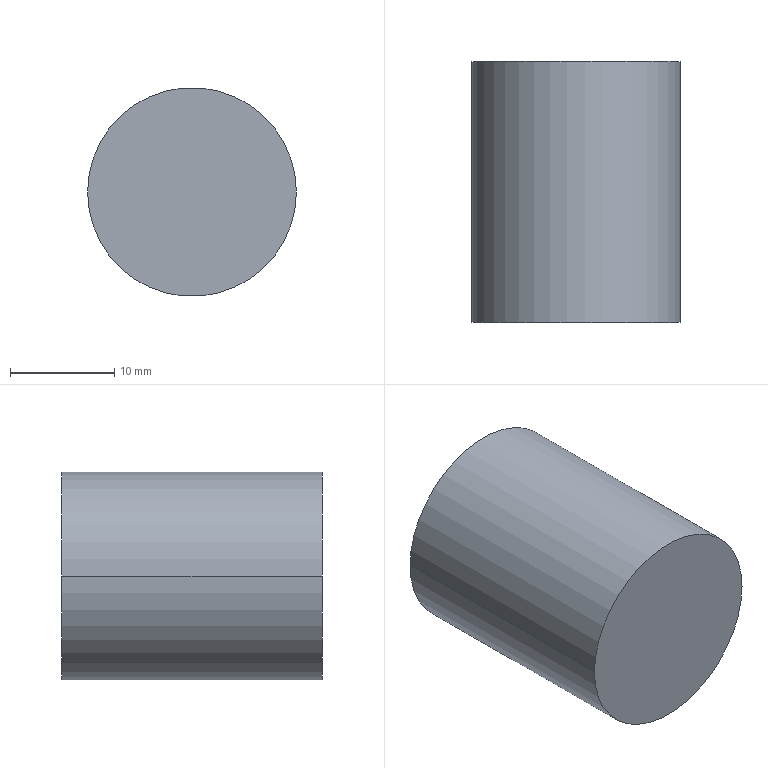Component | SolidWorks | LegSupport-1 | 1 solid | 4 faces | box 20 x 25 x 20 mm | volume 7854 mm3 | cylinder 2 | plane 2 | commonest cylinder face diameters 20 x2
build123d program:
from build123d import *

# Parameters (mm, degrees)
SKETCH1_R           = 10
BOSS_EXTRUDE1_DEPTH = 25


with BuildPart() as part:
    # Sketch1 → Boss-Extrude1 (new body)
    with BuildSketch(Plane.XY):
        with Locations((-290.265, 54.821)):
            Circle(SKETCH1_R)
    extrude(amount=BOSS_EXTRUDE1_DEPTH)


solid = part.part

# Placed as in the assembly
solid = solid.moved(Location((-81.735, 185, -108.821), (90, 0, 0)))
STEP:
#1=COLOUR_RGB('',0.7922,0.8196,0.9333);
#2=FILL_AREA_STYLE_COLOUR('',#1);
#3=FILL_AREA_STYLE('',(#2));
#4=SURFACE_STYLE_FILL_AREA(#3);
#5=SURFACE_SIDE_STYLE('',(#4));
#6=SURFACE_STYLE_USAGE(.BOTH.,#5);
#7=PRESENTATION_STYLE_ASSIGNMENT((#6));
#8=CARTESIAN_POINT('',(-14.252,7.283,-2.126));
#9=VERTEX_POINT('',#8);
#10=CARTESIAN_POINT('',(-15.039,7.283,-2.126));
#11=VERTEX_POINT('',#10);
#12=CARTESIAN_POINT('',(-14.646,7.283,-2.126));
#13=DIRECTION('',(0.,1.,0.));
#14=DIRECTION('',(1.,0.,0.));
#15=AXIS2_PLACEMENT_3D('',#12,#13,#14);
#16=CIRCLE('',#15,0.3937);
#17=EDGE_CURVE('',#9,#11,#16,.T.);
#18=ORIENTED_EDGE('',*,*,#17,.F.);
#19=CARTESIAN_POINT('',(-14.252,6.299,-2.126));
#20=VERTEX_POINT('',#19);
#21=CARTESIAN_POINT('',(-14.252,7.283,-2.126));
#22=DIRECTION('',(0.,-1.,0.));
#23=VECTOR('',#22,39.37);
#24=LINE('',#21,#23);
#25=EDGE_CURVE('',#9,#20,#24,.T.);
#26=ORIENTED_EDGE('',*,*,#25,.T.);
#27=CARTESIAN_POINT('',(-15.039,6.299,-2.126));
#28=VERTEX_POINT('',#27);
#29=CARTESIAN_POINT('',(-14.646,6.299,-2.126));
#30=DIRECTION('',(0.,1.,0.));
#31=DIRECTION('',(1.,0.,0.));
#32=AXIS2_PLACEMENT_3D('',#29,#30,#31);
#33=CIRCLE('',#32,0.3937);
#34=EDGE_CURVE('',#20,#28,#33,.T.);
#35=ORIENTED_EDGE('',*,*,#34,.T.);
#36=CARTESIAN_POINT('',(-15.039,7.283,-2.126));
#37=DIRECTION('',(0.,-1.,0.));
#38=VECTOR('',#37,39.37);
#39=LINE('',#36,#38);
#40=EDGE_CURVE('',#11,#28,#39,.T.);
#41=ORIENTED_EDGE('',*,*,#40,.F.);
#42=EDGE_LOOP('',(#18,#26,#35,#41));
#43=FACE_OUTER_BOUND('',#42,.T.);
#44=CARTESIAN_POINT('',(-14.646,7.283,-2.126));
#45=DIRECTION('',(0.,-1.,0.));
#46=DIRECTION('',(-1.,0.,0.));
#47=AXIS2_PLACEMENT_3D('',#44,#45,#46);
#48=CYLINDRICAL_SURFACE('',#47,0.3937);
#49=ADVANCED_FACE('',(#43),#48,.T.);
#50=ORIENTED_EDGE('',*,*,#25,.F.);
#51=CARTESIAN_POINT('',(-14.646,7.283,-2.126));
#52=DIRECTION('',(0.,1.,0.));
#53=DIRECTION('',(1.,0.,0.));
#54=AXIS2_PLACEMENT_3D('',#51,#52,#53);
#55=CIRCLE('',#54,0.3937);
#56=EDGE_CURVE('',#11,#9,#55,.T.);
#57=ORIENTED_EDGE('',*,*,#56,.F.);
#58=ORIENTED_EDGE('',*,*,#40,.T.);
#59=CARTESIAN_POINT('',(-14.646,6.299,-2.126));
#60=DIRECTION('',(0.,1.,0.));
#61=DIRECTION('',(1.,0.,0.));
#62=AXIS2_PLACEMENT_3D('',#59,#60,#61);
#63=CIRCLE('',#62,0.3937);
#64=EDGE_CURVE('',#28,#20,#63,.T.);
#65=ORIENTED_EDGE('',*,*,#64,.T.);
#66=EDGE_LOOP('',(#50,#57,#58,#65));
#67=FACE_OUTER_BOUND('',#66,.T.);
#68=CARTESIAN_POINT('',(-14.646,7.283,-2.126));
#69=DIRECTION('',(0.,-1.,0.));
#70=DIRECTION('',(-1.,0.,0.));
#71=AXIS2_PLACEMENT_3D('',#68,#69,#70);
#72=CYLINDRICAL_SURFACE('',#71,0.3937);
#73=ADVANCED_FACE('',(#67),#72,.T.);
#74=ORIENTED_EDGE('',*,*,#56,.T.);
#75=ORIENTED_EDGE('',*,*,#17,.T.);
#76=EDGE_LOOP('',(#74,#75));
#77=FACE_OUTER_BOUND('',#76,.T.);
#78=CARTESIAN_POINT('',(-14.646,7.283,-2.126));
#79=DIRECTION('',(0.,1.,0.));
#80=DIRECTION('',(1.,0.,0.));
#81=AXIS2_PLACEMENT_3D('',#78,#79,#80);
#82=PLANE('',#81);
#83=ADVANCED_FACE('',(#77),#82,.T.);
#84=ORIENTED_EDGE('',*,*,#64,.F.);
#85=ORIENTED_EDGE('',*,*,#34,.F.);
#86=EDGE_LOOP('',(#84,#85));
#87=FACE_OUTER_BOUND('',#86,.T.);
#88=CARTESIAN_POINT('',(-14.646,6.299,-2.126));
#89=DIRECTION('',(0.,1.,0.));
#90=DIRECTION('',(1.,0.,0.));
#91=AXIS2_PLACEMENT_3D('',#88,#89,#90);
#92=PLANE('',#91);
#93=ADVANCED_FACE('',(#87),#92,.F.);
#94=CLOSED_SHELL('',(#49,#73,#83,#93));
#95=MANIFOLD_SOLID_BREP('',#94);
#96=STYLED_ITEM('',(#7),#95);
#97=PRESENTATION_LAYER_ASSIGNMENT('','',(#96));
#98=(LENGTH_UNIT()NAMED_UNIT(*)SI_UNIT($,.METRE.));
#99=LENGTH_MEASURE_WITH_UNIT(LENGTH_MEASURE(0.0254),#98);
#100=DIMENSIONAL_EXPONENTS(1.,0.,0.,0.,0.,0.,0.);
#101=(CONVERSION_BASED_UNIT('',#99)LENGTH_UNIT()NAMED_UNIT(#100));
#102=UNCERTAINTY_MEASURE_WITH_UNIT(LENGTH_MEASURE(0.00001),#101,'','');
#103=(NAMED_UNIT(*)PLANE_ANGLE_UNIT()SI_UNIT($,.RADIAN.));
#104=(NAMED_UNIT(*)SI_UNIT($,.STERADIAN.)SOLID_ANGLE_UNIT());
#105=(GEOMETRIC_REPRESENTATION_CONTEXT(3)GLOBAL_UNCERTAINTY_ASSIGNED_CONTEXT((#102))GLOBAL_UNIT_ASSIGNED_CONTEXT((#101,#103,#104))REPRESENTATION_CONTEXT('',''));
#106=MECHANICAL_DESIGN_GEOMETRIC_PRESENTATION_REPRESENTATION('',(#96),#105);
#107=CARTESIAN_POINT('',(0.,0.,0.));
#108=DIRECTION('',(0.,0.,1.));
#109=DIRECTION('',(1.,0.,0.));
#110=AXIS2_PLACEMENT_3D('',#107,#108,#109);
#111=(LENGTH_UNIT()NAMED_UNIT(*)SI_UNIT($,.METRE.));
#112=LENGTH_MEASURE_WITH_UNIT(LENGTH_MEASURE(0.0254),#111);
#113=DIMENSIONAL_EXPONENTS(1.,0.,0.,0.,0.,0.,0.);
#114=(CONVERSION_BASED_UNIT('',#112)LENGTH_UNIT()NAMED_UNIT(#113));
#115=UNCERTAINTY_MEASURE_WITH_UNIT(LENGTH_MEASURE(0.00001),#114,'','');
#116=(NAMED_UNIT(*)PLANE_ANGLE_UNIT()SI_UNIT($,.RADIAN.));
#117=(NAMED_UNIT(*)SI_UNIT($,.STERADIAN.)SOLID_ANGLE_UNIT());
#118=(GEOMETRIC_REPRESENTATION_CONTEXT(3)GLOBAL_UNCERTAINTY_ASSIGNED_CONTEXT((#115))GLOBAL_UNIT_ASSIGNED_CONTEXT((#114,#116,#117))REPRESENTATION_CONTEXT('',''));
#119=ADVANCED_BREP_SHAPE_REPRESENTATION('',(#95,#110),#118);